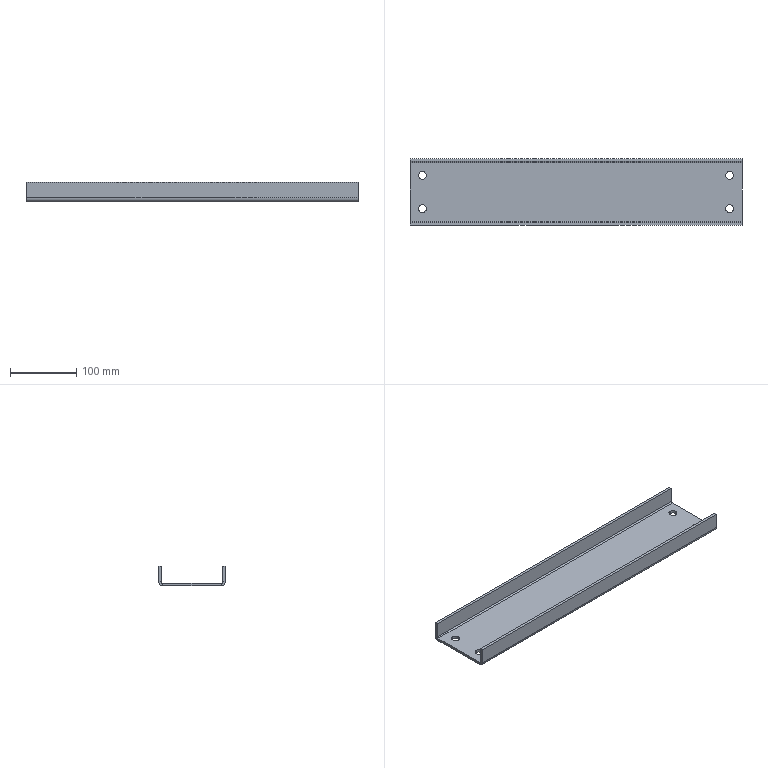Component | SolidWorks | JGS02-0001LegTieRod2-1 | 1 solid | 30 faces | box 500 x 100 x 30 mm | volume 295323 mm3 | plane 18 | cylinder 12 | commonest cylinder face diameters 12 x10 4 x2 | material Plain Carbon Steel
STEP:
#1=CARTESIAN_POINT('',(-5.674,-6.678,11.846));
#2=VERTEX_POINT('',#1);
#3=CARTESIAN_POINT('',(-5.674,-7.151,11.846));
#4=VERTEX_POINT('',#3);
#5=CARTESIAN_POINT('',(-5.674,-6.915,11.846));
#6=DIRECTION('',(0.,0.,-1.));
#7=DIRECTION('',(0.,-1.,0.));
#8=AXIS2_PLACEMENT_3D('',#5,#6,#7);
#9=CIRCLE('',#8,0.2362);
#10=EDGE_CURVE('',#2,#4,#9,.T.);
#11=ORIENTED_EDGE('',*,*,#10,.F.);
#12=CARTESIAN_POINT('',(-5.674,-6.678,11.689));
#13=VERTEX_POINT('',#12);
#14=CARTESIAN_POINT('',(-5.674,-6.678,11.846));
#15=DIRECTION('',(0.,0.,-1.));
#16=VECTOR('',#15,39.37);
#17=LINE('',#14,#16);
#18=EDGE_CURVE('',#2,#13,#17,.T.);
#19=ORIENTED_EDGE('',*,*,#18,.T.);
#20=CARTESIAN_POINT('',(-5.674,-7.151,11.689));
#21=VERTEX_POINT('',#20);
#22=CARTESIAN_POINT('',(-5.674,-6.915,11.689));
#23=DIRECTION('',(0.,0.,-1.));
#24=DIRECTION('',(0.,-1.,0.));
#25=AXIS2_PLACEMENT_3D('',#22,#23,#24);
#26=CIRCLE('',#25,0.2362);
#27=EDGE_CURVE('',#13,#21,#26,.T.);
#28=ORIENTED_EDGE('',*,*,#27,.T.);
#29=CARTESIAN_POINT('',(-5.674,-7.151,11.846));
#30=DIRECTION('',(0.,0.,-1.));
#31=VECTOR('',#30,39.37);
#32=LINE('',#29,#31);
#33=EDGE_CURVE('',#4,#21,#32,.T.);
#34=ORIENTED_EDGE('',*,*,#33,.F.);
#35=EDGE_LOOP('',(#11,#19,#28,#34));
#36=FACE_OUTER_BOUND('',#35,.T.);
#37=CARTESIAN_POINT('',(-5.674,-6.915,11.846));
#38=DIRECTION('',(0.,0.,-1.));
#39=DIRECTION('',(0.,-1.,0.));
#40=AXIS2_PLACEMENT_3D('',#37,#38,#39);
#41=CYLINDRICAL_SURFACE('',#40,0.2362);
#42=ADVANCED_FACE('',(#36),#41,.F.);
#43=CARTESIAN_POINT('',(-5.674,-4.71,11.846));
#44=VERTEX_POINT('',#43);
#45=CARTESIAN_POINT('',(-5.674,-5.182,11.846));
#46=VERTEX_POINT('',#45);
#47=CARTESIAN_POINT('',(-5.674,-4.946,11.846));
#48=DIRECTION('',(0.,0.,-1.));
#49=DIRECTION('',(0.,-1.,0.));
#50=AXIS2_PLACEMENT_3D('',#47,#48,#49);
#51=CIRCLE('',#50,0.2362);
#52=EDGE_CURVE('',#44,#46,#51,.T.);
#53=ORIENTED_EDGE('',*,*,#52,.F.);
#54=CARTESIAN_POINT('',(-5.674,-4.71,11.689));
#55=VERTEX_POINT('',#54);
#56=CARTESIAN_POINT('',(-5.674,-4.71,11.846));
#57=DIRECTION('',(0.,0.,-1.));
#58=VECTOR('',#57,39.37);
#59=LINE('',#56,#58);
#60=EDGE_CURVE('',#44,#55,#59,.T.);
#61=ORIENTED_EDGE('',*,*,#60,.T.);
#62=CARTESIAN_POINT('',(-5.674,-5.182,11.689));
#63=VERTEX_POINT('',#62);
#64=CARTESIAN_POINT('',(-5.674,-4.946,11.689));
#65=DIRECTION('',(0.,0.,-1.));
#66=DIRECTION('',(0.,-1.,0.));
#67=AXIS2_PLACEMENT_3D('',#64,#65,#66);
#68=CIRCLE('',#67,0.2362);
#69=EDGE_CURVE('',#55,#63,#68,.T.);
#70=ORIENTED_EDGE('',*,*,#69,.T.);
#71=CARTESIAN_POINT('',(-5.674,-5.182,11.846));
#72=DIRECTION('',(0.,0.,-1.));
#73=VECTOR('',#72,39.37);
#74=LINE('',#71,#73);
#75=EDGE_CURVE('',#46,#63,#74,.T.);
#76=ORIENTED_EDGE('',*,*,#75,.F.);
#77=EDGE_LOOP('',(#53,#61,#70,#76));
#78=FACE_OUTER_BOUND('',#77,.T.);
#79=CARTESIAN_POINT('',(-5.674,-4.946,11.846));
#80=DIRECTION('',(0.,0.,-1.));
#81=DIRECTION('',(0.,-1.,0.));
#82=AXIS2_PLACEMENT_3D('',#79,#80,#81);
#83=CYLINDRICAL_SURFACE('',#82,0.2362);
#84=ADVANCED_FACE('',(#78),#83,.F.);
#85=CARTESIAN_POINT('',(12.554,-6.678,11.846));
#86=VERTEX_POINT('',#85);
#87=CARTESIAN_POINT('',(12.554,-7.151,11.846));
#88=VERTEX_POINT('',#87);
#89=CARTESIAN_POINT('',(12.554,-6.915,11.846));
#90=DIRECTION('',(0.,0.,-1.));
#91=DIRECTION('',(0.,-1.,0.));
#92=AXIS2_PLACEMENT_3D('',#89,#90,#91);
#93=CIRCLE('',#92,0.2362);
#94=EDGE_CURVE('',#86,#88,#93,.T.);
#95=ORIENTED_EDGE('',*,*,#94,.F.);
#96=CARTESIAN_POINT('',(12.554,-6.678,11.689));
#97=VERTEX_POINT('',#96);
#98=CARTESIAN_POINT('',(12.554,-6.678,11.846));
#99=DIRECTION('',(0.,0.,-1.));
#100=VECTOR('',#99,39.37);
#101=LINE('',#98,#100);
#102=EDGE_CURVE('',#86,#97,#101,.T.);
#103=ORIENTED_EDGE('',*,*,#102,.T.);
#104=CARTESIAN_POINT('',(12.554,-7.151,11.689));
#105=VERTEX_POINT('',#104);
#106=CARTESIAN_POINT('',(12.554,-6.915,11.689));
#107=DIRECTION('',(0.,0.,-1.));
#108=DIRECTION('',(0.,-1.,0.));
#109=AXIS2_PLACEMENT_3D('',#106,#107,#108);
#110=CIRCLE('',#109,0.2362);
#111=EDGE_CURVE('',#97,#105,#110,.T.);
#112=ORIENTED_EDGE('',*,*,#111,.T.);
#113=CARTESIAN_POINT('',(12.554,-7.151,11.846));
#114=DIRECTION('',(0.,0.,-1.));
#115=VECTOR('',#114,39.37);
#116=LINE('',#113,#115);
#117=EDGE_CURVE('',#88,#105,#116,.T.);
#118=ORIENTED_EDGE('',*,*,#117,.F.);
#119=EDGE_LOOP('',(#95,#103,#112,#118));
#120=FACE_OUTER_BOUND('',#119,.T.);
#121=CARTESIAN_POINT('',(12.554,-6.915,11.846));
#122=DIRECTION('',(0.,0.,-1.));
#123=DIRECTION('',(0.,-1.,0.));
#124=AXIS2_PLACEMENT_3D('',#121,#122,#123);
#125=CYLINDRICAL_SURFACE('',#124,0.2362);
#126=ADVANCED_FACE('',(#120),#125,.F.);
#127=CARTESIAN_POINT('',(12.554,-4.71,11.846));
#128=VERTEX_POINT('',#127);
#129=CARTESIAN_POINT('',(12.554,-5.182,11.846));
#130=VERTEX_POINT('',#129);
#131=CARTESIAN_POINT('',(12.554,-4.946,11.846));
#132=DIRECTION('',(0.,0.,-1.));
#133=DIRECTION('',(0.,-1.,0.));
#134=AXIS2_PLACEMENT_3D('',#131,#132,#133);
#135=CIRCLE('',#134,0.2362);
#136=EDGE_CURVE('',#128,#130,#135,.T.);
#137=ORIENTED_EDGE('',*,*,#136,.F.);
#138=CARTESIAN_POINT('',(12.554,-4.71,11.689));
#139=VERTEX_POINT('',#138);
#140=CARTESIAN_POINT('',(12.554,-4.71,11.846));
#141=DIRECTION('',(0.,0.,-1.));
#142=VECTOR('',#141,39.37);
#143=LINE('',#140,#142);
#144=EDGE_CURVE('',#128,#139,#143,.T.);
#145=ORIENTED_EDGE('',*,*,#144,.T.);
#146=CARTESIAN_POINT('',(12.554,-5.182,11.689));
#147=VERTEX_POINT('',#146);
#148=CARTESIAN_POINT('',(12.554,-4.946,11.689));
#149=DIRECTION('',(0.,0.,-1.));
#150=DIRECTION('',(0.,-1.,0.));
#151=AXIS2_PLACEMENT_3D('',#148,#149,#150);
#152=CIRCLE('',#151,0.2362);
#153=EDGE_CURVE('',#139,#147,#152,.T.);
#154=ORIENTED_EDGE('',*,*,#153,.T.);
#155=CARTESIAN_POINT('',(12.554,-5.182,11.846));
#156=DIRECTION('',(0.,0.,-1.));
#157=VECTOR('',#156,39.37);
#158=LINE('',#155,#157);
#159=EDGE_CURVE('',#130,#147,#158,.T.);
#160=ORIENTED_EDGE('',*,*,#159,.F.);
#161=EDGE_LOOP('',(#137,#145,#154,#160));
#162=FACE_OUTER_BOUND('',#161,.T.);
#163=CARTESIAN_POINT('',(12.554,-4.946,11.846));
#164=DIRECTION('',(0.,0.,-1.));
#165=DIRECTION('',(0.,-1.,0.));
#166=AXIS2_PLACEMENT_3D('',#163,#164,#165);
#167=CYLINDRICAL_SURFACE('',#166,0.2362);
#168=ADVANCED_FACE('',(#162),#167,.F.);
#169=CARTESIAN_POINT('',(-6.402,-3.962,11.925));
#170=VERTEX_POINT('',#169);
#171=CARTESIAN_POINT('',(-6.402,-4.119,11.925));
#172=VERTEX_POINT('',#171);
#173=CARTESIAN_POINT('',(-6.402,-3.962,11.925));
#174=DIRECTION('',(0.,-1.,-0.));
#175=VECTOR('',#174,39.37);
#176=LINE('',#173,#175);
#177=EDGE_CURVE('',#170,#172,#176,.T.);
#178=ORIENTED_EDGE('',*,*,#177,.F.);
#179=CARTESIAN_POINT('',(-6.402,-4.198,11.689));
#180=VERTEX_POINT('',#179);
#181=CARTESIAN_POINT('',(-6.402,-4.198,11.925));
#182=DIRECTION('',(-1.,-0.,-0.));
#183=DIRECTION('',(0.,0.,-1.));
#184=AXIS2_PLACEMENT_3D('',#181,#182,#183);
#185=CIRCLE('',#184,0.2362);
#186=EDGE_CURVE('',#170,#180,#185,.T.);
#187=ORIENTED_EDGE('',*,*,#186,.T.);
#188=CARTESIAN_POINT('',(-6.402,-4.198,11.846));
#189=VERTEX_POINT('',#188);
#190=CARTESIAN_POINT('',(-6.402,-4.198,11.846));
#191=DIRECTION('',(0.,0.,-1.));
#192=VECTOR('',#191,39.37);
#193=LINE('',#190,#192);
#194=EDGE_CURVE('',#189,#180,#193,.T.);
#195=ORIENTED_EDGE('',*,*,#194,.F.);
#196=CARTESIAN_POINT('',(-6.402,-4.198,11.925));
#197=DIRECTION('',(-1.,-0.,-0.));
#198=DIRECTION('',(0.,0.,1.));
#199=AXIS2_PLACEMENT_3D('',#196,#197,#198);
#200=CIRCLE('',#199,0.07874);
#201=EDGE_CURVE('',#172,#189,#200,.T.);
#202=ORIENTED_EDGE('',*,*,#201,.F.);
#203=EDGE_LOOP('',(#178,#187,#195,#202));
#204=FACE_OUTER_BOUND('',#203,.T.);
#205=CARTESIAN_POINT('',(-6.402,-3.962,11.925));
#206=DIRECTION('',(-1.,-0.,-0.));
#207=DIRECTION('',(-0.,-0.,1.));
#208=AXIS2_PLACEMENT_3D('',#205,#206,#207);
#209=PLANE('',#208);
#210=ADVANCED_FACE('',(#204),#209,.T.);
#211=CARTESIAN_POINT('',(-6.402,-3.962,12.87));
#212=VERTEX_POINT('',#211);
#213=CARTESIAN_POINT('',(-6.402,-3.962,11.689));
#214=DIRECTION('',(0.,0.,-1.));
#215=VECTOR('',#214,39.37);
#216=LINE('',#213,#215);
#217=EDGE_CURVE('',#212,#170,#216,.T.);
#218=ORIENTED_EDGE('',*,*,#217,.T.);
#219=ORIENTED_EDGE('',*,*,#177,.T.);
#220=CARTESIAN_POINT('',(-6.402,-4.119,12.87));
#221=VERTEX_POINT('',#220);
#222=CARTESIAN_POINT('',(-6.402,-4.119,11.689));
#223=DIRECTION('',(0.,0.,-1.));
#224=VECTOR('',#223,39.37);
#225=LINE('',#222,#224);
#226=EDGE_CURVE('',#221,#172,#225,.T.);
#227=ORIENTED_EDGE('',*,*,#226,.F.);
#228=CARTESIAN_POINT('',(-6.402,-3.962,12.87));
#229=DIRECTION('',(0.,-1.,0.));
#230=VECTOR('',#229,39.37);
#231=LINE('',#228,#230);
#232=EDGE_CURVE('',#212,#221,#231,.T.);
#233=ORIENTED_EDGE('',*,*,#232,.F.);
#234=EDGE_LOOP('',(#218,#219,#227,#233));
#235=FACE_OUTER_BOUND('',#234,.T.);
#236=CARTESIAN_POINT('',(-6.402,-4.198,11.846));
#237=DIRECTION('',(-1.,-0.,-0.));
#238=DIRECTION('',(-0.,-0.,1.));
#239=AXIS2_PLACEMENT_3D('',#236,#237,#238);
#240=PLANE('',#239);
#241=ADVANCED_FACE('',(#235),#240,.T.);
#242=CARTESIAN_POINT('',(13.283,-4.198,11.689));
#243=VERTEX_POINT('',#242);
#244=CARTESIAN_POINT('',(13.283,-4.198,11.846));
#245=VERTEX_POINT('',#244);
#246=CARTESIAN_POINT('',(13.283,-4.198,11.689));
#247=DIRECTION('',(-0.,-0.,1.));
#248=VECTOR('',#247,39.37);
#249=LINE('',#246,#248);
#250=EDGE_CURVE('',#243,#245,#249,.T.);
#251=ORIENTED_EDGE('',*,*,#250,.F.);
#252=CARTESIAN_POINT('',(13.283,-3.962,11.925));
#253=VERTEX_POINT('',#252);
#254=CARTESIAN_POINT('',(13.283,-4.198,11.925));
#255=DIRECTION('',(-1.,-0.,-0.));
#256=DIRECTION('',(0.,0.,-1.));
#257=AXIS2_PLACEMENT_3D('',#254,#255,#256);
#258=CIRCLE('',#257,0.2362);
#259=EDGE_CURVE('',#253,#243,#258,.T.);
#260=ORIENTED_EDGE('',*,*,#259,.F.);
#261=CARTESIAN_POINT('',(13.283,-4.119,11.925));
#262=VERTEX_POINT('',#261);
#263=CARTESIAN_POINT('',(13.283,-4.119,11.925));
#264=DIRECTION('',(-0.,1.,0.));
#265=VECTOR('',#264,39.37);
#266=LINE('',#263,#265);
#267=EDGE_CURVE('',#262,#253,#266,.T.);
#268=ORIENTED_EDGE('',*,*,#267,.F.);
#269=CARTESIAN_POINT('',(13.283,-4.198,11.925));
#270=DIRECTION('',(-1.,-0.,-0.));
#271=DIRECTION('',(0.,0.,1.));
#272=AXIS2_PLACEMENT_3D('',#269,#270,#271);
#273=CIRCLE('',#272,0.07874);
#274=EDGE_CURVE('',#262,#245,#273,.T.);
#275=ORIENTED_EDGE('',*,*,#274,.T.);
#276=EDGE_LOOP('',(#251,#260,#268,#275));
#277=FACE_OUTER_BOUND('',#276,.T.);
#278=CARTESIAN_POINT('',(13.283,-4.198,11.689));
#279=DIRECTION('',(1.,0.,0.));
#280=DIRECTION('',(0.,0.,-1.));
#281=AXIS2_PLACEMENT_3D('',#278,#279,#280);
#282=PLANE('',#281);
#283=ADVANCED_FACE('',(#277),#282,.T.);
#284=CARTESIAN_POINT('',(13.283,-7.663,11.689));
#285=VERTEX_POINT('',#284);
#286=CARTESIAN_POINT('',(13.283,-3.962,11.689));
#287=DIRECTION('',(0.,-1.,0.));
#288=VECTOR('',#287,39.37);
#289=LINE('',#286,#288);
#290=EDGE_CURVE('',#243,#285,#289,.T.);
#291=ORIENTED_EDGE('',*,*,#290,.F.);
#292=ORIENTED_EDGE('',*,*,#250,.T.);
#293=CARTESIAN_POINT('',(13.283,-7.663,11.846));
#294=VERTEX_POINT('',#293);
#295=CARTESIAN_POINT('',(13.283,-3.962,11.846));
#296=DIRECTION('',(0.,-1.,0.));
#297=VECTOR('',#296,39.37);
#298=LINE('',#295,#297);
#299=EDGE_CURVE('',#245,#294,#298,.T.);
#300=ORIENTED_EDGE('',*,*,#299,.T.);
#301=CARTESIAN_POINT('',(13.283,-7.663,11.846));
#302=DIRECTION('',(0.,0.,-1.));
#303=VECTOR('',#302,39.37);
#304=LINE('',#301,#303);
#305=EDGE_CURVE('',#294,#285,#304,.T.);
#306=ORIENTED_EDGE('',*,*,#305,.T.);
#307=EDGE_LOOP('',(#291,#292,#300,#306));
#308=FACE_OUTER_BOUND('',#307,.T.);
#309=CARTESIAN_POINT('',(13.283,-4.119,11.925));
#310=DIRECTION('',(1.,0.,0.));
#311=DIRECTION('',(0.,0.,-1.));
#312=AXIS2_PLACEMENT_3D('',#309,#310,#311);
#313=PLANE('',#312);
#314=ADVANCED_FACE('',(#308),#313,.T.);
#315=CARTESIAN_POINT('',(-6.402,-7.663,11.689));
#316=VERTEX_POINT('',#315);
#317=CARTESIAN_POINT('',(-6.402,-7.663,11.846));
#318=VERTEX_POINT('',#317);
#319=CARTESIAN_POINT('',(-6.402,-7.663,11.689));
#320=DIRECTION('',(-0.,-0.,1.));
#321=VECTOR('',#320,39.37);
#322=LINE('',#319,#321);
#323=EDGE_CURVE('',#316,#318,#322,.T.);
#324=ORIENTED_EDGE('',*,*,#323,.F.);
#325=CARTESIAN_POINT('',(-6.402,-7.899,11.925));
#326=VERTEX_POINT('',#325);
#327=CARTESIAN_POINT('',(-6.402,-7.663,11.925));
#328=DIRECTION('',(-1.,-0.,-0.));
#329=DIRECTION('',(0.,0.,-1.));
#330=AXIS2_PLACEMENT_3D('',#327,#328,#329);
#331=CIRCLE('',#330,0.2362);
#332=EDGE_CURVE('',#316,#326,#331,.T.);
#333=ORIENTED_EDGE('',*,*,#332,.T.);
#334=CARTESIAN_POINT('',(-6.402,-7.741,11.925));
#335=VERTEX_POINT('',#334);
#336=CARTESIAN_POINT('',(-6.402,-7.741,11.925));
#337=DIRECTION('',(0.,-1.,-0.));
#338=VECTOR('',#337,39.37);
#339=LINE('',#336,#338);
#340=EDGE_CURVE('',#335,#326,#339,.T.);
#341=ORIENTED_EDGE('',*,*,#340,.F.);
#342=CARTESIAN_POINT('',(-6.402,-7.663,11.925));
#343=DIRECTION('',(-1.,-0.,-0.));
#344=DIRECTION('',(0.,0.,1.));
#345=AXIS2_PLACEMENT_3D('',#342,#343,#344);
#346=CIRCLE('',#345,0.07874);
#347=EDGE_CURVE('',#318,#335,#346,.T.);
#348=ORIENTED_EDGE('',*,*,#347,.F.);
#349=EDGE_LOOP('',(#324,#333,#341,#348));
#350=FACE_OUTER_BOUND('',#349,.T.);
#351=CARTESIAN_POINT('',(-6.402,-7.663,11.689));
#352=DIRECTION('',(-1.,-0.,-0.));
#353=DIRECTION('',(-0.,-0.,1.));
#354=AXIS2_PLACEMENT_3D('',#351,#352,#353);
#355=PLANE('',#354);
#356=ADVANCED_FACE('',(#350),#355,.T.);
#357=CARTESIAN_POINT('',(-6.402,-3.962,11.689));
#358=DIRECTION('',(0.,-1.,0.));
#359=VECTOR('',#358,39.37);
#360=LINE('',#357,#359);
#361=EDGE_CURVE('',#180,#316,#360,.T.);
#362=ORIENTED_EDGE('',*,*,#361,.T.);
#363=ORIENTED_EDGE('',*,*,#323,.T.);
#364=CARTESIAN_POINT('',(-6.402,-3.962,11.846));
#365=DIRECTION('',(0.,-1.,0.));
#366=VECTOR('',#365,39.37);
#367=LINE('',#364,#366);
#368=EDGE_CURVE('',#189,#318,#367,.T.);
#369=ORIENTED_EDGE('',*,*,#368,.F.);
#370=ORIENTED_EDGE('',*,*,#194,.T.);
#371=EDGE_LOOP('',(#362,#363,#369,#370));
#372=FACE_OUTER_BOUND('',#371,.T.);
#373=CARTESIAN_POINT('',(-6.402,-7.741,11.925));
#374=DIRECTION('',(-1.,-0.,-0.));
#375=DIRECTION('',(-0.,-0.,1.));
#376=AXIS2_PLACEMENT_3D('',#373,#374,#375);
#377=PLANE('',#376);
#378=ADVANCED_FACE('',(#372),#377,.T.);
#379=CARTESIAN_POINT('',(13.283,-7.899,11.925));
#380=VERTEX_POINT('',#379);
#381=CARTESIAN_POINT('',(13.283,-7.741,11.925));
#382=VERTEX_POINT('',#381);
#383=CARTESIAN_POINT('',(13.283,-7.899,11.925));
#384=DIRECTION('',(-0.,1.,0.));
#385=VECTOR('',#384,39.37);
#386=LINE('',#383,#385);
#387=EDGE_CURVE('',#380,#382,#386,.T.);
#388=ORIENTED_EDGE('',*,*,#387,.F.);
#389=CARTESIAN_POINT('',(13.283,-7.663,11.925));
#390=DIRECTION('',(-1.,-0.,-0.));
#391=DIRECTION('',(0.,0.,-1.));
#392=AXIS2_PLACEMENT_3D('',#389,#390,#391);
#393=CIRCLE('',#392,0.2362);
#394=EDGE_CURVE('',#285,#380,#393,.T.);
#395=ORIENTED_EDGE('',*,*,#394,.F.);
#396=ORIENTED_EDGE('',*,*,#305,.F.);
#397=CARTESIAN_POINT('',(13.283,-7.663,11.925));
#398=DIRECTION('',(-1.,-0.,-0.));
#399=DIRECTION('',(0.,0.,1.));
#400=AXIS2_PLACEMENT_3D('',#397,#398,#399);
#401=CIRCLE('',#400,0.07874);
#402=EDGE_CURVE('',#294,#382,#401,.T.);
#403=ORIENTED_EDGE('',*,*,#402,.T.);
#404=EDGE_LOOP('',(#388,#395,#396,#403));
#405=FACE_OUTER_BOUND('',#404,.T.);
#406=CARTESIAN_POINT('',(13.283,-7.899,11.925));
#407=DIRECTION('',(1.,0.,0.));
#408=DIRECTION('',(0.,0.,-1.));
#409=AXIS2_PLACEMENT_3D('',#406,#407,#408);
#410=PLANE('',#409);
#411=ADVANCED_FACE('',(#405),#410,.T.);
#412=CARTESIAN_POINT('',(13.283,-7.899,12.87));
#413=VERTEX_POINT('',#412);
#414=CARTESIAN_POINT('',(13.283,-7.899,11.689));
#415=DIRECTION('',(-0.,-0.,1.));
#416=VECTOR('',#415,39.37);
#417=LINE('',#414,#416);
#418=EDGE_CURVE('',#380,#413,#417,.T.);
#419=ORIENTED_EDGE('',*,*,#418,.F.);
#420=ORIENTED_EDGE('',*,*,#387,.T.);
#421=CARTESIAN_POINT('',(13.283,-7.741,12.87));
#422=VERTEX_POINT('',#421);
#423=CARTESIAN_POINT('',(13.283,-7.741,11.689));
#424=DIRECTION('',(-0.,-0.,1.));
#425=VECTOR('',#424,39.37);
#426=LINE('',#423,#425);
#427=EDGE_CURVE('',#382,#422,#426,.T.);
#428=ORIENTED_EDGE('',*,*,#427,.T.);
#429=CARTESIAN_POINT('',(13.283,-7.741,12.87));
#430=DIRECTION('',(0.,-1.,-0.));
#431=VECTOR('',#430,39.37);
#432=LINE('',#429,#431);
#433=EDGE_CURVE('',#422,#413,#432,.T.);
#434=ORIENTED_EDGE('',*,*,#433,.T.);
#435=EDGE_LOOP('',(#419,#420,#428,#434));
#436=FACE_OUTER_BOUND('',#435,.T.);
#437=CARTESIAN_POINT('',(13.283,-7.663,11.846));
#438=DIRECTION('',(1.,0.,0.));
#439=DIRECTION('',(0.,0.,-1.));
#440=AXIS2_PLACEMENT_3D('',#437,#438,#439);
#441=PLANE('',#440);
#442=ADVANCED_FACE('',(#436),#441,.T.);
#443=ORIENTED_EDGE('',*,*,#418,.T.);
#444=CARTESIAN_POINT('',(-6.402,-7.899,12.87));
#445=VERTEX_POINT('',#444);
#446=CARTESIAN_POINT('',(-6.402,-7.899,12.87));
#447=DIRECTION('',(1.,0.,0.));
#448=VECTOR('',#447,39.37);
#449=LINE('',#446,#448);
#450=EDGE_CURVE('',#445,#413,#449,.T.);
#451=ORIENTED_EDGE('',*,*,#450,.F.);
#452=CARTESIAN_POINT('',(-6.402,-7.899,11.689));
#453=DIRECTION('',(-0.,-0.,1.));
#454=VECTOR('',#453,39.37);
#455=LINE('',#452,#454);
#456=EDGE_CURVE('',#326,#445,#455,.T.);
#457=ORIENTED_EDGE('',*,*,#456,.F.);
#458=CARTESIAN_POINT('',(-6.402,-7.899,11.925));
#459=DIRECTION('',(1.,0.,0.));
#460=VECTOR('',#459,39.37);
#461=LINE('',#458,#460);
#462=EDGE_CURVE('',#326,#380,#461,.T.);
#463=ORIENTED_EDGE('',*,*,#462,.T.);
#464=EDGE_LOOP('',(#443,#451,#457,#463));
#465=FACE_OUTER_BOUND('',#464,.T.);
#466=CARTESIAN_POINT('',(-6.402,-7.899,11.689));
#467=DIRECTION('',(-0.,1.,0.));
#468=DIRECTION('',(0.,0.,-1.));
#469=AXIS2_PLACEMENT_3D('',#466,#467,#468);
#470=PLANE('',#469);
#471=ADVANCED_FACE('',(#465),#470,.F.);
#472=ORIENTED_EDGE('',*,*,#433,.F.);
#473=CARTESIAN_POINT('',(-6.402,-7.741,12.87));
#474=VERTEX_POINT('',#473);
#475=CARTESIAN_POINT('',(-6.402,-7.741,12.87));
#476=DIRECTION('',(1.,0.,0.));
#477=VECTOR('',#476,39.37);
#478=LINE('',#475,#477);
#479=EDGE_CURVE('',#474,#422,#478,.T.);
#480=ORIENTED_EDGE('',*,*,#479,.F.);
#481=CARTESIAN_POINT('',(-6.402,-7.741,12.87));
#482=DIRECTION('',(0.,-1.,-0.));
#483=VECTOR('',#482,39.37);
#484=LINE('',#481,#483);
#485=EDGE_CURVE('',#474,#445,#484,.T.);
#486=ORIENTED_EDGE('',*,*,#485,.T.);
#487=ORIENTED_EDGE('',*,*,#450,.T.);
#488=EDGE_LOOP('',(#472,#480,#486,#487));
#489=FACE_OUTER_BOUND('',#488,.T.);
#490=CARTESIAN_POINT('',(-6.402,-7.741,12.87));
#491=DIRECTION('',(-0.,-0.,1.));
#492=DIRECTION('',(1.,0.,0.));
#493=AXIS2_PLACEMENT_3D('',#490,#491,#492);
#494=PLANE('',#493);
#495=ADVANCED_FACE('',(#489),#494,.T.);
#496=ORIENTED_EDGE('',*,*,#427,.F.);
#497=CARTESIAN_POINT('',(-6.402,-7.741,11.925));
#498=DIRECTION('',(1.,0.,0.));
#499=VECTOR('',#498,39.37);
#500=LINE('',#497,#499);
#501=EDGE_CURVE('',#335,#382,#500,.T.);
#502=ORIENTED_EDGE('',*,*,#501,.F.);
#503=CARTESIAN_POINT('',(-6.402,-7.741,11.689));
#504=DIRECTION('',(-0.,-0.,1.));
#505=VECTOR('',#504,39.37);
#506=LINE('',#503,#505);
#507=EDGE_CURVE('',#335,#474,#506,.T.);
#508=ORIENTED_EDGE('',*,*,#507,.T.);
#509=ORIENTED_EDGE('',*,*,#479,.T.);
#510=EDGE_LOOP('',(#496,#502,#508,#509));
#511=FACE_OUTER_BOUND('',#510,.T.);
#512=CARTESIAN_POINT('',(-6.402,-7.741,11.689));
#513=DIRECTION('',(-0.,1.,0.));
#514=DIRECTION('',(0.,0.,-1.));
#515=AXIS2_PLACEMENT_3D('',#512,#513,#514);
#516=PLANE('',#515);
#517=ADVANCED_FACE('',(#511),#516,.T.);
#518=ORIENTED_EDGE('',*,*,#402,.F.);
#519=CARTESIAN_POINT('',(-6.402,-7.663,11.846));
#520=DIRECTION('',(1.,0.,0.));
#521=VECTOR('',#520,39.37);
#522=LINE('',#519,#521);
#523=EDGE_CURVE('',#318,#294,#522,.T.);
#524=ORIENTED_EDGE('',*,*,#523,.F.);
#525=ORIENTED_EDGE('',*,*,#347,.T.);
#526=ORIENTED_EDGE('',*,*,#501,.T.);
#527=EDGE_LOOP('',(#518,#524,#525,#526));
#528=FACE_OUTER_BOUND('',#527,.T.);
#529=CARTESIAN_POINT('',(-6.402,-7.663,11.925));
#530=DIRECTION('',(1.,0.,0.));
#531=DIRECTION('',(0.,0.,-1.));
#532=AXIS2_PLACEMENT_3D('',#529,#530,#531);
#533=CYLINDRICAL_SURFACE('',#532,0.07874);
#534=ADVANCED_FACE('',(#528),#533,.F.);
#535=CARTESIAN_POINT('',(-5.674,-6.915,11.846));
#536=DIRECTION('',(0.,0.,-1.));
#537=DIRECTION('',(0.,-1.,0.));
#538=AXIS2_PLACEMENT_3D('',#535,#536,#537);
#539=CIRCLE('',#538,0.2362);
#540=EDGE_CURVE('',#4,#2,#539,.T.);
#541=ORIENTED_EDGE('',*,*,#540,.T.);
#542=ORIENTED_EDGE('',*,*,#10,.T.);
#543=EDGE_LOOP('',(#541,#542));
#544=FACE_BOUND('',#543,.T.);
#545=CARTESIAN_POINT('',(-5.674,-4.946,11.846));
#546=DIRECTION('',(0.,0.,-1.));
#547=DIRECTION('',(0.,-1.,0.));
#548=AXIS2_PLACEMENT_3D('',#545,#546,#547);
#549=CIRCLE('',#548,0.2362);
#550=EDGE_CURVE('',#46,#44,#549,.T.);
#551=ORIENTED_EDGE('',*,*,#550,.T.);
#552=ORIENTED_EDGE('',*,*,#52,.T.);
#553=EDGE_LOOP('',(#551,#552));
#554=FACE_BOUND('',#553,.T.);
#555=CARTESIAN_POINT('',(12.554,-6.915,11.846));
#556=DIRECTION('',(0.,0.,-1.));
#557=DIRECTION('',(0.,-1.,0.));
#558=AXIS2_PLACEMENT_3D('',#555,#556,#557);
#559=CIRCLE('',#558,0.2362);
#560=EDGE_CURVE('',#88,#86,#559,.T.);
#561=ORIENTED_EDGE('',*,*,#560,.T.);
#562=ORIENTED_EDGE('',*,*,#94,.T.);
#563=EDGE_LOOP('',(#561,#562));
#564=FACE_BOUND('',#563,.T.);
#565=CARTESIAN_POINT('',(12.554,-4.946,11.846));
#566=DIRECTION('',(0.,0.,-1.));
#567=DIRECTION('',(0.,-1.,0.));
#568=AXIS2_PLACEMENT_3D('',#565,#566,#567);
#569=CIRCLE('',#568,0.2362);
#570=EDGE_CURVE('',#130,#128,#569,.T.);
#571=ORIENTED_EDGE('',*,*,#570,.T.);
#572=ORIENTED_EDGE('',*,*,#136,.T.);
#573=EDGE_LOOP('',(#571,#572));
#574=FACE_BOUND('',#573,.T.);
#575=ORIENTED_EDGE('',*,*,#299,.F.);
#576=CARTESIAN_POINT('',(-6.402,-4.198,11.846));
#577=DIRECTION('',(1.,0.,0.));
#578=VECTOR('',#577,39.37);
#579=LINE('',#576,#578);
#580=EDGE_CURVE('',#189,#245,#579,.T.);
#581=ORIENTED_EDGE('',*,*,#580,.F.);
#582=ORIENTED_EDGE('',*,*,#368,.T.);
#583=ORIENTED_EDGE('',*,*,#523,.T.);
#584=EDGE_LOOP('',(#575,#581,#582,#583));
#585=FACE_OUTER_BOUND('',#584,.T.);
#586=CARTESIAN_POINT('',(-6.402,-3.962,11.846));
#587=DIRECTION('',(-0.,-0.,1.));
#588=DIRECTION('',(-0.,1.,-0.));
#589=AXIS2_PLACEMENT_3D('',#586,#587,#588);
#590=PLANE('',#589);
#591=ADVANCED_FACE('',(#544,#554,#564,#574,#585),#590,.T.);
#592=ORIENTED_EDGE('',*,*,#274,.F.);
#593=CARTESIAN_POINT('',(-6.402,-4.119,11.925));
#594=DIRECTION('',(1.,0.,0.));
#595=VECTOR('',#594,39.37);
#596=LINE('',#593,#595);
#597=EDGE_CURVE('',#172,#262,#596,.T.);
#598=ORIENTED_EDGE('',*,*,#597,.F.);
#599=ORIENTED_EDGE('',*,*,#201,.T.);
#600=ORIENTED_EDGE('',*,*,#580,.T.);
#601=EDGE_LOOP('',(#592,#598,#599,#600));
#602=FACE_OUTER_BOUND('',#601,.T.);
#603=CARTESIAN_POINT('',(-6.402,-4.198,11.925));
#604=DIRECTION('',(1.,0.,0.));
#605=DIRECTION('',(0.,0.,-1.));
#606=AXIS2_PLACEMENT_3D('',#603,#604,#605);
#607=CYLINDRICAL_SURFACE('',#606,0.07874);
#608=ADVANCED_FACE('',(#602),#607,.F.);
#609=CARTESIAN_POINT('',(13.283,-4.119,12.87));
#610=VERTEX_POINT('',#609);
#611=CARTESIAN_POINT('',(13.283,-4.119,11.689));
#612=DIRECTION('',(0.,0.,-1.));
#613=VECTOR('',#612,39.37);
#614=LINE('',#611,#613);
#615=EDGE_CURVE('',#610,#262,#614,.T.);
#616=ORIENTED_EDGE('',*,*,#615,.F.);
#617=CARTESIAN_POINT('',(-6.402,-4.119,12.87));
#618=DIRECTION('',(1.,0.,0.));
#619=VECTOR('',#618,39.37);
#620=LINE('',#617,#619);
#621=EDGE_CURVE('',#221,#610,#620,.T.);
#622=ORIENTED_EDGE('',*,*,#621,.F.);
#623=ORIENTED_EDGE('',*,*,#226,.T.);
#624=ORIENTED_EDGE('',*,*,#597,.T.);
#625=EDGE_LOOP('',(#616,#622,#623,#624));
#626=FACE_OUTER_BOUND('',#625,.T.);
#627=CARTESIAN_POINT('',(-6.402,-4.119,11.689));
#628=DIRECTION('',(0.,-1.,-0.));
#629=DIRECTION('',(-0.,-0.,1.));
#630=AXIS2_PLACEMENT_3D('',#627,#628,#629);
#631=PLANE('',#630);
#632=ADVANCED_FACE('',(#626),#631,.T.);
#633=CARTESIAN_POINT('',(13.283,-3.962,12.87));
#634=VERTEX_POINT('',#633);
#635=CARTESIAN_POINT('',(13.283,-3.962,12.87));
#636=DIRECTION('',(0.,-1.,0.));
#637=VECTOR('',#636,39.37);
#638=LINE('',#635,#637);
#639=EDGE_CURVE('',#634,#610,#638,.T.);
#640=ORIENTED_EDGE('',*,*,#639,.F.);
#641=CARTESIAN_POINT('',(-6.402,-3.962,12.87));
#642=DIRECTION('',(1.,0.,0.));
#643=VECTOR('',#642,39.37);
#644=LINE('',#641,#643);
#645=EDGE_CURVE('',#212,#634,#644,.T.);
#646=ORIENTED_EDGE('',*,*,#645,.F.);
#647=ORIENTED_EDGE('',*,*,#232,.T.);
#648=ORIENTED_EDGE('',*,*,#621,.T.);
#649=EDGE_LOOP('',(#640,#646,#647,#648));
#650=FACE_OUTER_BOUND('',#649,.T.);
#651=CARTESIAN_POINT('',(-6.402,-3.962,12.87));
#652=DIRECTION('',(-0.,0.,1.));
#653=DIRECTION('',(-0.,1.,-0.));
#654=AXIS2_PLACEMENT_3D('',#651,#652,#653);
#655=PLANE('',#654);
#656=ADVANCED_FACE('',(#650),#655,.T.);
#657=CARTESIAN_POINT('',(13.283,-3.962,11.689));
#658=DIRECTION('',(0.,0.,-1.));
#659=VECTOR('',#658,39.37);
#660=LINE('',#657,#659);
#661=EDGE_CURVE('',#634,#253,#660,.T.);
#662=ORIENTED_EDGE('',*,*,#661,.T.);
#663=CARTESIAN_POINT('',(-6.402,-3.962,11.925));
#664=DIRECTION('',(1.,0.,0.));
#665=VECTOR('',#664,39.37);
#666=LINE('',#663,#665);
#667=EDGE_CURVE('',#170,#253,#666,.T.);
#668=ORIENTED_EDGE('',*,*,#667,.F.);
#669=ORIENTED_EDGE('',*,*,#217,.F.);
#670=ORIENTED_EDGE('',*,*,#645,.T.);
#671=EDGE_LOOP('',(#662,#668,#669,#670));
#672=FACE_OUTER_BOUND('',#671,.T.);
#673=CARTESIAN_POINT('',(-6.402,-3.962,11.689));
#674=DIRECTION('',(0.,-1.,-0.));
#675=DIRECTION('',(-0.,-0.,1.));
#676=AXIS2_PLACEMENT_3D('',#673,#674,#675);
#677=PLANE('',#676);
#678=ADVANCED_FACE('',(#672),#677,.F.);
#679=ORIENTED_EDGE('',*,*,#259,.T.);
#680=CARTESIAN_POINT('',(-6.402,-4.198,11.689));
#681=DIRECTION('',(1.,0.,0.));
#682=VECTOR('',#681,39.37);
#683=LINE('',#680,#682);
#684=EDGE_CURVE('',#180,#243,#683,.T.);
#685=ORIENTED_EDGE('',*,*,#684,.F.);
#686=ORIENTED_EDGE('',*,*,#186,.F.);
#687=ORIENTED_EDGE('',*,*,#667,.T.);
#688=EDGE_LOOP('',(#679,#685,#686,#687));
#689=FACE_OUTER_BOUND('',#688,.T.);
#690=CARTESIAN_POINT('',(-6.402,-4.198,11.925));
#691=DIRECTION('',(1.,0.,0.));
#692=DIRECTION('',(0.,0.,-1.));
#693=AXIS2_PLACEMENT_3D('',#690,#691,#692);
#694=CYLINDRICAL_SURFACE('',#693,0.2362);
#695=ADVANCED_FACE('',(#689),#694,.T.);
#696=CARTESIAN_POINT('',(-5.674,-6.915,11.689));
#697=DIRECTION('',(0.,0.,-1.));
#698=DIRECTION('',(0.,-1.,0.));
#699=AXIS2_PLACEMENT_3D('',#696,#697,#698);
#700=CIRCLE('',#699,0.2362);
#701=EDGE_CURVE('',#21,#13,#700,.T.);
#702=ORIENTED_EDGE('',*,*,#701,.F.);
#703=ORIENTED_EDGE('',*,*,#27,.F.);
#704=EDGE_LOOP('',(#702,#703));
#705=FACE_BOUND('',#704,.T.);
#706=CARTESIAN_POINT('',(-5.674,-4.946,11.689));
#707=DIRECTION('',(0.,0.,-1.));
#708=DIRECTION('',(0.,-1.,0.));
#709=AXIS2_PLACEMENT_3D('',#706,#707,#708);
#710=CIRCLE('',#709,0.2362);
#711=EDGE_CURVE('',#63,#55,#710,.T.);
#712=ORIENTED_EDGE('',*,*,#711,.F.);
#713=ORIENTED_EDGE('',*,*,#69,.F.);
#714=EDGE_LOOP('',(#712,#713));
#715=FACE_BOUND('',#714,.T.);
#716=CARTESIAN_POINT('',(12.554,-6.915,11.689));
#717=DIRECTION('',(0.,0.,-1.));
#718=DIRECTION('',(0.,-1.,0.));
#719=AXIS2_PLACEMENT_3D('',#716,#717,#718);
#720=CIRCLE('',#719,0.2362);
#721=EDGE_CURVE('',#105,#97,#720,.T.);
#722=ORIENTED_EDGE('',*,*,#721,.F.);
#723=ORIENTED_EDGE('',*,*,#111,.F.);
#724=EDGE_LOOP('',(#722,#723));
#725=FACE_BOUND('',#724,.T.);
#726=CARTESIAN_POINT('',(12.554,-4.946,11.689));
#727=DIRECTION('',(0.,0.,-1.));
#728=DIRECTION('',(0.,-1.,0.));
#729=AXIS2_PLACEMENT_3D('',#726,#727,#728);
#730=CIRCLE('',#729,0.2362);
#731=EDGE_CURVE('',#147,#139,#730,.T.);
#732=ORIENTED_EDGE('',*,*,#731,.F.);
#733=ORIENTED_EDGE('',*,*,#153,.F.);
#734=EDGE_LOOP('',(#732,#733));
#735=FACE_BOUND('',#734,.T.);
#736=ORIENTED_EDGE('',*,*,#290,.T.);
#737=CARTESIAN_POINT('',(-6.402,-7.663,11.689));
#738=DIRECTION('',(1.,0.,0.));
#739=VECTOR('',#738,39.37);
#740=LINE('',#737,#739);
#741=EDGE_CURVE('',#316,#285,#740,.T.);
#742=ORIENTED_EDGE('',*,*,#741,.F.);
#743=ORIENTED_EDGE('',*,*,#361,.F.);
#744=ORIENTED_EDGE('',*,*,#684,.T.);
#745=EDGE_LOOP('',(#736,#742,#743,#744));
#746=FACE_OUTER_BOUND('',#745,.T.);
#747=CARTESIAN_POINT('',(-6.402,-3.962,11.689));
#748=DIRECTION('',(-0.,-0.,1.));
#749=DIRECTION('',(-0.,1.,-0.));
#750=AXIS2_PLACEMENT_3D('',#747,#748,#749);
#751=PLANE('',#750);
#752=ADVANCED_FACE('',(#705,#715,#725,#735,#746),#751,.F.);
#753=ORIENTED_EDGE('',*,*,#394,.T.);
#754=ORIENTED_EDGE('',*,*,#462,.F.);
#755=ORIENTED_EDGE('',*,*,#332,.F.);
#756=ORIENTED_EDGE('',*,*,#741,.T.);
#757=EDGE_LOOP('',(#753,#754,#755,#756));
#758=FACE_OUTER_BOUND('',#757,.T.);
#759=CARTESIAN_POINT('',(-6.402,-7.663,11.925));
#760=DIRECTION('',(1.,0.,0.));
#761=DIRECTION('',(0.,0.,-1.));
#762=AXIS2_PLACEMENT_3D('',#759,#760,#761);
#763=CYLINDRICAL_SURFACE('',#762,0.2362);
#764=ADVANCED_FACE('',(#758),#763,.T.);
#765=ORIENTED_EDGE('',*,*,#456,.T.);
#766=ORIENTED_EDGE('',*,*,#485,.F.);
#767=ORIENTED_EDGE('',*,*,#507,.F.);
#768=ORIENTED_EDGE('',*,*,#340,.T.);
#769=EDGE_LOOP('',(#765,#766,#767,#768));
#770=FACE_OUTER_BOUND('',#769,.T.);
#771=CARTESIAN_POINT('',(-6.402,-7.663,11.925));
#772=DIRECTION('',(-1.,-0.,-0.));
#773=DIRECTION('',(-0.,-0.,1.));
#774=AXIS2_PLACEMENT_3D('',#771,#772,#773);
#775=PLANE('',#774);
#776=ADVANCED_FACE('',(#770),#775,.T.);
#777=ORIENTED_EDGE('',*,*,#615,.T.);
#778=ORIENTED_EDGE('',*,*,#267,.T.);
#779=ORIENTED_EDGE('',*,*,#661,.F.);
#780=ORIENTED_EDGE('',*,*,#639,.T.);
#781=EDGE_LOOP('',(#777,#778,#779,#780));
#782=FACE_OUTER_BOUND('',#781,.T.);
#783=CARTESIAN_POINT('',(13.283,-7.663,11.925));
#784=DIRECTION('',(-1.,-0.,-0.));
#785=DIRECTION('',(-0.,-0.,1.));
#786=AXIS2_PLACEMENT_3D('',#783,#784,#785);
#787=PLANE('',#786);
#788=ADVANCED_FACE('',(#782),#787,.F.);
#789=ORIENTED_EDGE('',*,*,#144,.F.);
#790=ORIENTED_EDGE('',*,*,#570,.F.);
#791=ORIENTED_EDGE('',*,*,#159,.T.);
#792=ORIENTED_EDGE('',*,*,#731,.T.);
#793=EDGE_LOOP('',(#789,#790,#791,#792));
#794=FACE_OUTER_BOUND('',#793,.T.);
#795=CARTESIAN_POINT('',(12.554,-4.946,11.846));
#796=DIRECTION('',(0.,0.,-1.));
#797=DIRECTION('',(0.,-1.,0.));
#798=AXIS2_PLACEMENT_3D('',#795,#796,#797);
#799=CYLINDRICAL_SURFACE('',#798,0.2362);
#800=ADVANCED_FACE('',(#794),#799,.F.);
#801=ORIENTED_EDGE('',*,*,#102,.F.);
#802=ORIENTED_EDGE('',*,*,#560,.F.);
#803=ORIENTED_EDGE('',*,*,#117,.T.);
#804=ORIENTED_EDGE('',*,*,#721,.T.);
#805=EDGE_LOOP('',(#801,#802,#803,#804));
#806=FACE_OUTER_BOUND('',#805,.T.);
#807=CARTESIAN_POINT('',(12.554,-6.915,11.846));
#808=DIRECTION('',(0.,0.,-1.));
#809=DIRECTION('',(0.,-1.,0.));
#810=AXIS2_PLACEMENT_3D('',#807,#808,#809);
#811=CYLINDRICAL_SURFACE('',#810,0.2362);
#812=ADVANCED_FACE('',(#806),#811,.F.);
#813=ORIENTED_EDGE('',*,*,#60,.F.);
#814=ORIENTED_EDGE('',*,*,#550,.F.);
#815=ORIENTED_EDGE('',*,*,#75,.T.);
#816=ORIENTED_EDGE('',*,*,#711,.T.);
#817=EDGE_LOOP('',(#813,#814,#815,#816));
#818=FACE_OUTER_BOUND('',#817,.T.);
#819=CARTESIAN_POINT('',(-5.674,-4.946,11.846));
#820=DIRECTION('',(0.,0.,-1.));
#821=DIRECTION('',(0.,-1.,0.));
#822=AXIS2_PLACEMENT_3D('',#819,#820,#821);
#823=CYLINDRICAL_SURFACE('',#822,0.2362);
#824=ADVANCED_FACE('',(#818),#823,.F.);
#825=ORIENTED_EDGE('',*,*,#18,.F.);
#826=ORIENTED_EDGE('',*,*,#540,.F.);
#827=ORIENTED_EDGE('',*,*,#33,.T.);
#828=ORIENTED_EDGE('',*,*,#701,.T.);
#829=EDGE_LOOP('',(#825,#826,#827,#828));
#830=FACE_OUTER_BOUND('',#829,.T.);
#831=CARTESIAN_POINT('',(-5.674,-6.915,11.846));
#832=DIRECTION('',(0.,0.,-1.));
#833=DIRECTION('',(0.,-1.,0.));
#834=AXIS2_PLACEMENT_3D('',#831,#832,#833);
#835=CYLINDRICAL_SURFACE('',#834,0.2362);
#836=ADVANCED_FACE('',(#830),#835,.F.);
#837=CLOSED_SHELL('',(#42,#84,#126,#168,#210,#241,#283,#314,#356,#378,#411,#442,#471,#495,#517,#534,#591,#608,#632,#656,#678,#695,#752,#764,#776,#788,#800,#812,#824,#836));
#838=MANIFOLD_SOLID_BREP('',#837);
#839=CARTESIAN_POINT('',(0.,0.,0.));
#840=DIRECTION('',(0.,0.,1.));
#841=DIRECTION('',(1.,0.,0.));
#842=AXIS2_PLACEMENT_3D('',#839,#840,#841);
#843=(LENGTH_UNIT()NAMED_UNIT(*)SI_UNIT($,.METRE.));
#844=LENGTH_MEASURE_WITH_UNIT(LENGTH_MEASURE(0.0254),#843);
#845=DIMENSIONAL_EXPONENTS(1.,0.,0.,0.,0.,0.,0.);
#846=(CONVERSION_BASED_UNIT('',#844)LENGTH_UNIT()NAMED_UNIT(#845));
#847=UNCERTAINTY_MEASURE_WITH_UNIT(LENGTH_MEASURE(0.00001),#846,'','');
#848=(NAMED_UNIT(*)PLANE_ANGLE_UNIT()SI_UNIT($,.RADIAN.));
#849=(NAMED_UNIT(*)SI_UNIT($,.STERADIAN.)SOLID_ANGLE_UNIT());
#850=(GEOMETRIC_REPRESENTATION_CONTEXT(3)GLOBAL_UNCERTAINTY_ASSIGNED_CONTEXT((#847))GLOBAL_UNIT_ASSIGNED_CONTEXT((#846,#848,#849))REPRESENTATION_CONTEXT('',''));
#851=ADVANCED_BREP_SHAPE_REPRESENTATION('',(#838,#842),#850);
#852=COLOUR_RGB('',0.7922,0.8196,0.9333);
#853=FILL_AREA_STYLE_COLOUR('',#852);
#854=FILL_AREA_STYLE('',(#853));
#855=SURFACE_STYLE_FILL_AREA(#854);
#856=SURFACE_SIDE_STYLE('',(#855));
#857=SURFACE_STYLE_USAGE(.BOTH.,#856);
#858=PRESENTATION_STYLE_ASSIGNMENT((#857));
#859=STYLED_ITEM('',(#858),#838);
#860=(LENGTH_UNIT()NAMED_UNIT(*)SI_UNIT($,.METRE.));
#861=LENGTH_MEASURE_WITH_UNIT(LENGTH_MEASURE(0.0254),#860);
#862=DIMENSIONAL_EXPONENTS(1.,0.,0.,0.,0.,0.,0.);
#863=(CONVERSION_BASED_UNIT('',#861)LENGTH_UNIT()NAMED_UNIT(#862));
#864=UNCERTAINTY_MEASURE_WITH_UNIT(LENGTH_MEASURE(0.00001),#863,'','');
#865=(NAMED_UNIT(*)PLANE_ANGLE_UNIT()SI_UNIT($,.RADIAN.));
#866=(NAMED_UNIT(*)SI_UNIT($,.STERADIAN.)SOLID_ANGLE_UNIT());
#867=(GEOMETRIC_REPRESENTATION_CONTEXT(3)GLOBAL_UNCERTAINTY_ASSIGNED_CONTEXT((#864))GLOBAL_UNIT_ASSIGNED_CONTEXT((#863,#865,#866))REPRESENTATION_CONTEXT('',''));
#868=MECHANICAL_DESIGN_GEOMETRIC_PRESENTATION_REPRESENTATION('',(#859),#867);
#869=PRESENTATION_LAYER_ASSIGNMENT('','',(#859));